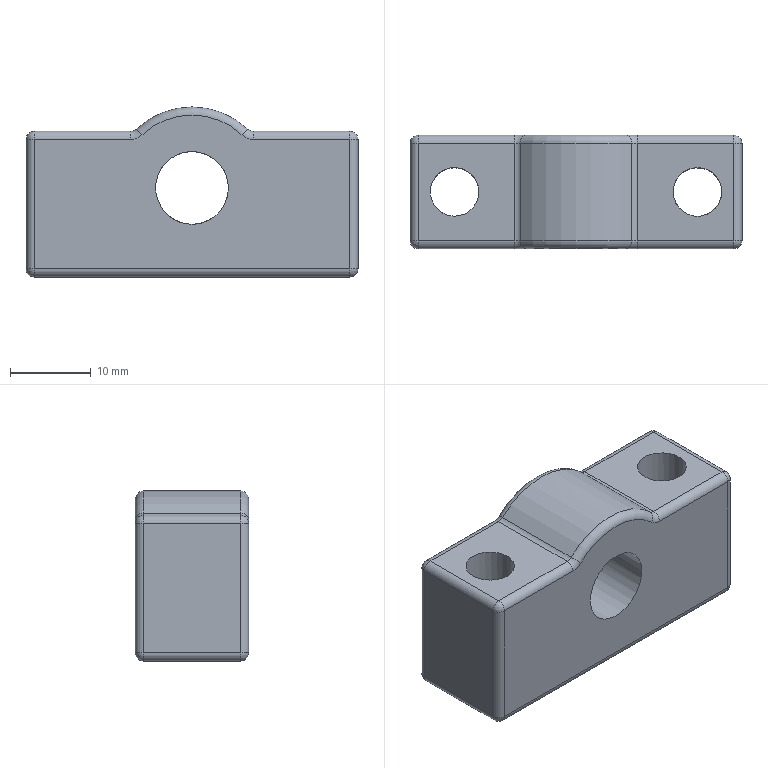Component | NX | BRACKET_3 | 1 solid | 41 faces | volume 8776 mm3 | cylinder 20 | sphere 8 | plane 7 | torus 6 | commonest cylinder face diameters 2 x16 6 x2 20 x1 9 x1